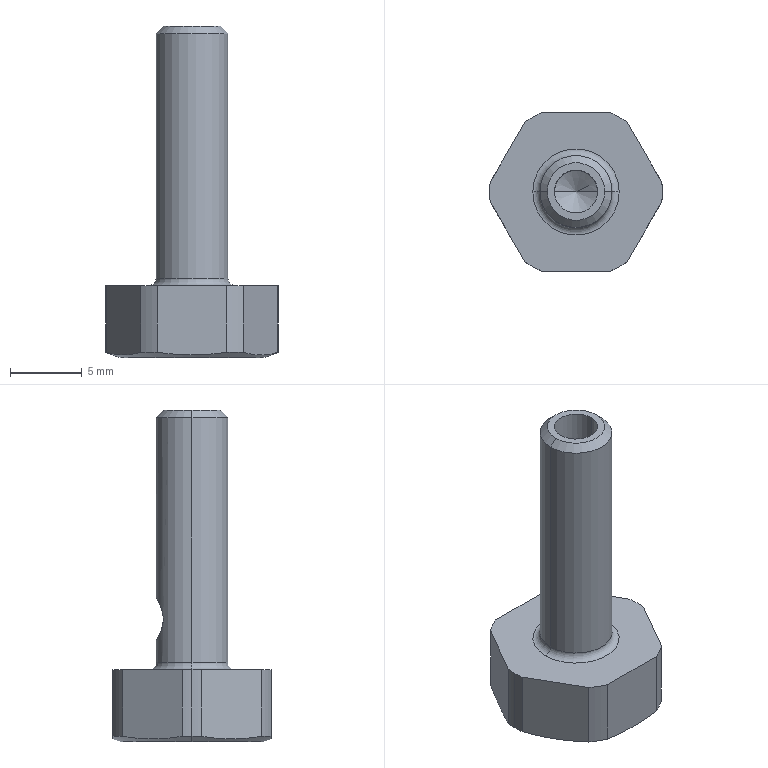Component | SolidWorks | 6.11-1937032107-0-2 | 1 solid | 32 faces | box 12 x 11 x 23 mm | volume 743 mm3 | cylinder 15 | plane 9 | cone 6 | torus 2 | commonest cylinder face diameters 12 x7 3 x6 5 x2 | material 40Cr
STEP:
#1=CARTESIAN_POINT('',(-0.09843,-1.772,-2.067));
#2=VERTEX_POINT('',#1);
#3=CARTESIAN_POINT('',(0.09843,-1.772,-2.067));
#4=VERTEX_POINT('',#3);
#5=CARTESIAN_POINT('',(0.,-1.772,-2.067));
#6=DIRECTION('',(0.,0.,1.));
#7=DIRECTION('',(1.,0.,0.));
#8=AXIS2_PLACEMENT_3D('',#5,#6,#7);
#9=CIRCLE('',#8,0.09843);
#10=EDGE_CURVE('',#2,#4,#9,.T.);
#11=ORIENTED_EDGE('',*,*,#10,.F.);
#12=CARTESIAN_POINT('',(-0.1181,-1.772,-2.087));
#13=VERTEX_POINT('',#12);
#14=CARTESIAN_POINT('',(-0.1181,-1.772,-2.067));
#15=DIRECTION('',(0.,1.,0.));
#16=DIRECTION('',(-1.,0.,0.));
#17=AXIS2_PLACEMENT_3D('',#14,#15,#16);
#18=CIRCLE('',#17,0.01969);
#19=EDGE_CURVE('',#2,#13,#18,.T.);
#20=ORIENTED_EDGE('',*,*,#19,.T.);
#21=CARTESIAN_POINT('',(0.1181,-1.772,-2.087));
#22=VERTEX_POINT('',#21);
#23=CARTESIAN_POINT('',(0.,-1.772,-2.087));
#24=DIRECTION('',(0.,0.,-1.));
#25=DIRECTION('',(1.,0.,0.));
#26=AXIS2_PLACEMENT_3D('',#23,#24,#25);
#27=CIRCLE('',#26,0.1181);
#28=EDGE_CURVE('',#22,#13,#27,.T.);
#29=ORIENTED_EDGE('',*,*,#28,.F.);
#30=CARTESIAN_POINT('',(0.1181,-1.772,-2.067));
#31=DIRECTION('',(0.,-1.,0.));
#32=DIRECTION('',(0.,0.,-1.));
#33=AXIS2_PLACEMENT_3D('',#30,#31,#32);
#34=CIRCLE('',#33,0.01969);
#35=EDGE_CURVE('',#4,#22,#34,.T.);
#36=ORIENTED_EDGE('',*,*,#35,.F.);
#37=EDGE_LOOP('',(#11,#20,#29,#36));
#38=FACE_OUTER_BOUND('',#37,.T.);
#39=CARTESIAN_POINT('',(0.,-1.772,-2.067));
#40=DIRECTION('',(0.,0.,1.));
#41=DIRECTION('',(1.,0.,0.));
#42=AXIS2_PLACEMENT_3D('',#39,#40,#41);
#43=TOROIDAL_SURFACE('',#42,0.1181,0.01969);
#44=ADVANCED_FACE('',(#38),#43,.F.);
#45=CARTESIAN_POINT('',(0.,-1.673,-1.89));
#46=VERTEX_POINT('',#45);
#47=CARTESIAN_POINT('',(0.,-1.673,-2.008));
#48=VERTEX_POINT('',#47);
#49=CARTESIAN_POINT('',(0.,-1.673,-1.89));
#50=CARTESIAN_POINT('',(-0.003988,-1.673,-1.89));
#51=CARTESIAN_POINT('',(-0.00791,-1.673,-1.89));
#52=CARTESIAN_POINT('',(-0.01563,-1.674,-1.892));
#53=CARTESIAN_POINT('',(-0.01942,-1.675,-1.893));
#54=CARTESIAN_POINT('',(-0.03011,-1.678,-1.897));
#55=CARTESIAN_POINT('',(-0.03651,-1.68,-1.902));
#56=CARTESIAN_POINT('',(-0.04449,-1.684,-1.91));
#57=CARTESIAN_POINT('',(-0.04691,-1.685,-1.913));
#58=CARTESIAN_POINT('',(-0.05111,-1.688,-1.919));
#59=CARTESIAN_POINT('',(-0.05291,-1.689,-1.922));
#60=CARTESIAN_POINT('',(-0.0559,-1.691,-1.929));
#61=CARTESIAN_POINT('',(-0.05707,-1.691,-1.933));
#62=CARTESIAN_POINT('',(-0.05864,-1.693,-1.941));
#63=CARTESIAN_POINT('',(-0.05905,-1.693,-1.945));
#64=CARTESIAN_POINT('',(-0.05906,-1.693,-1.957));
#65=CARTESIAN_POINT('',(-0.05742,-1.692,-1.965));
#66=CARTESIAN_POINT('',(-0.05294,-1.689,-1.975));
#67=CARTESIAN_POINT('',(-0.0511,-1.687,-1.979));
#68=CARTESIAN_POINT('',(-0.04688,-1.685,-1.985));
#69=CARTESIAN_POINT('',(-0.0445,-1.684,-1.988));
#70=CARTESIAN_POINT('',(-0.03645,-1.68,-1.996));
#71=CARTESIAN_POINT('',(-0.03014,-1.678,-2.));
#72=CARTESIAN_POINT('',(-0.0194,-1.675,-2.005));
#73=CARTESIAN_POINT('',(-0.01569,-1.674,-2.006));
#74=CARTESIAN_POINT('',(-0.00802,-1.673,-2.007));
#75=CARTESIAN_POINT('',(-0.004002,-1.673,-2.008));
#76=CARTESIAN_POINT('',(0.,-1.673,-2.008));
#77=B_SPLINE_CURVE_WITH_KNOTS('',3,(#49,#50,#51,#52,#53,#54,#55,#56,#57,#58,#59,#60,#61,#62,#63,#64,#65,#66,#67,#68,#69,#70,#71,#72,#73,#74,#75,#76),.UNSPECIFIED.,.F.,.F.,(4,2,2,2,2,2,2,2,2,2,2,2,2,4),(0.004812,0.005113,0.005413,0.006013,0.006313,0.006613,0.006914,0.007214,0.007814,0.008114,0.008415,0.009015,0.009315,0.009615),.UNSPECIFIED.);
#78=EDGE_CURVE('',#46,#48,#77,.T.);
#79=ORIENTED_EDGE('',*,*,#78,.F.);
#80=CARTESIAN_POINT('',(0.,-1.713,-1.89));
#81=VERTEX_POINT('',#80);
#82=CARTESIAN_POINT('',(0.,-1.772,-1.89));
#83=DIRECTION('',(0.,-1.,0.));
#84=VECTOR('',#83,39.37);
#85=LINE('',#82,#84);
#86=EDGE_CURVE('',#46,#81,#85,.T.);
#87=ORIENTED_EDGE('',*,*,#86,.T.);
#88=CARTESIAN_POINT('',(-0.05906,-1.772,-1.949));
#89=VERTEX_POINT('',#88);
#90=CARTESIAN_POINT('',(-0.05906,-1.772,-1.949));
#91=CARTESIAN_POINT('',(-0.05906,-1.737,-1.914));
#92=CARTESIAN_POINT('',(-0.03459,-1.713,-1.89));
#93=CARTESIAN_POINT('',(0.,-1.713,-1.89));
#94=(BOUNDED_CURVE()B_SPLINE_CURVE(3,(#90,#91,#92,#93),.UNSPECIFIED.,.F.,.F.)B_SPLINE_CURVE_WITH_KNOTS((4,4),(4.712,6.283),.UNSPECIFIED.)CURVE()GEOMETRIC_REPRESENTATION_ITEM()RATIONAL_B_SPLINE_CURVE((1.,0.8047,0.8047,1.))REPRESENTATION_ITEM(''));
#95=EDGE_CURVE('',#89,#81,#94,.T.);
#96=ORIENTED_EDGE('',*,*,#95,.F.);
#97=CARTESIAN_POINT('',(0.,-1.713,-2.008));
#98=VERTEX_POINT('',#97);
#99=CARTESIAN_POINT('',(0.,-1.713,-2.008));
#100=CARTESIAN_POINT('',(-0.03459,-1.713,-2.008));
#101=CARTESIAN_POINT('',(-0.05906,-1.737,-1.983));
#102=CARTESIAN_POINT('',(-0.05906,-1.772,-1.949));
#103=(BOUNDED_CURVE()B_SPLINE_CURVE(3,(#99,#100,#101,#102),.UNSPECIFIED.,.F.,.F.)B_SPLINE_CURVE_WITH_KNOTS((4,4),(3.142,4.712),.UNSPECIFIED.)CURVE()GEOMETRIC_REPRESENTATION_ITEM()RATIONAL_B_SPLINE_CURVE((1.,0.8047,0.8047,1.))REPRESENTATION_ITEM(''));
#104=EDGE_CURVE('',#98,#89,#103,.T.);
#105=ORIENTED_EDGE('',*,*,#104,.F.);
#106=CARTESIAN_POINT('',(0.,-1.772,-2.008));
#107=DIRECTION('',(0.,-1.,0.));
#108=VECTOR('',#107,39.37);
#109=LINE('',#106,#108);
#110=EDGE_CURVE('',#48,#98,#109,.T.);
#111=ORIENTED_EDGE('',*,*,#110,.F.);
#112=EDGE_LOOP('',(#79,#87,#96,#105,#111));
#113=FACE_OUTER_BOUND('',#112,.T.);
#114=CARTESIAN_POINT('',(0.,-1.772,-1.949));
#115=DIRECTION('',(0.,-1.,0.));
#116=DIRECTION('',(0.,0.,-1.));
#117=AXIS2_PLACEMENT_3D('',#114,#115,#116);
#118=CYLINDRICAL_SURFACE('',#117,0.05906);
#119=ADVANCED_FACE('',(#113),#118,.F.);
#120=CARTESIAN_POINT('',(-0.05906,-1.772,-2.008));
#121=VERTEX_POINT('',#120);
#122=CARTESIAN_POINT('',(0.05906,-1.772,-2.008));
#123=VERTEX_POINT('',#122);
#124=CARTESIAN_POINT('',(0.,-1.772,-2.008));
#125=DIRECTION('',(0.,0.,1.));
#126=DIRECTION('',(1.,0.,0.));
#127=AXIS2_PLACEMENT_3D('',#124,#125,#126);
#128=CIRCLE('',#127,0.05906);
#129=EDGE_CURVE('',#121,#123,#128,.T.);
#130=ORIENTED_EDGE('',*,*,#129,.F.);
#131=CARTESIAN_POINT('',(-0.05906,-1.772,-1.378));
#132=DIRECTION('',(0.,0.,1.));
#133=VECTOR('',#132,39.37);
#134=LINE('',#131,#133);
#135=EDGE_CURVE('',#121,#89,#134,.T.);
#136=ORIENTED_EDGE('',*,*,#135,.T.);
#137=CARTESIAN_POINT('',(-0.05906,-1.772,-1.378));
#138=VERTEX_POINT('',#137);
#139=CARTESIAN_POINT('',(-0.05906,-1.772,-1.378));
#140=DIRECTION('',(0.,0.,1.));
#141=VECTOR('',#140,39.37);
#142=LINE('',#139,#141);
#143=EDGE_CURVE('',#89,#138,#142,.T.);
#144=ORIENTED_EDGE('',*,*,#143,.T.);
#145=CARTESIAN_POINT('',(0.05906,-1.772,-1.378));
#146=VERTEX_POINT('',#145);
#147=CARTESIAN_POINT('',(0.,-1.772,-1.378));
#148=DIRECTION('',(0.,0.,1.));
#149=DIRECTION('',(1.,0.,0.));
#150=AXIS2_PLACEMENT_3D('',#147,#148,#149);
#151=CIRCLE('',#150,0.05906);
#152=EDGE_CURVE('',#138,#146,#151,.T.);
#153=ORIENTED_EDGE('',*,*,#152,.T.);
#154=CARTESIAN_POINT('',(0.05906,-1.772,-1.949));
#155=VERTEX_POINT('',#154);
#156=CARTESIAN_POINT('',(0.05906,-1.772,-1.378));
#157=DIRECTION('',(0.,0.,1.));
#158=VECTOR('',#157,39.37);
#159=LINE('',#156,#158);
#160=EDGE_CURVE('',#155,#146,#159,.T.);
#161=ORIENTED_EDGE('',*,*,#160,.F.);
#162=CARTESIAN_POINT('',(0.05906,-1.772,-1.378));
#163=DIRECTION('',(0.,0.,1.));
#164=VECTOR('',#163,39.37);
#165=LINE('',#162,#164);
#166=EDGE_CURVE('',#123,#155,#165,.T.);
#167=ORIENTED_EDGE('',*,*,#166,.F.);
#168=EDGE_LOOP('',(#130,#136,#144,#153,#161,#167));
#169=FACE_OUTER_BOUND('',#168,.T.);
#170=CARTESIAN_POINT('',(0.,-1.772,-1.378));
#171=DIRECTION('',(0.,0.,1.));
#172=DIRECTION('',(1.,0.,0.));
#173=AXIS2_PLACEMENT_3D('',#170,#171,#172);
#174=CYLINDRICAL_SURFACE('',#173,0.05906);
#175=ADVANCED_FACE('',(#169),#174,.F.);
#176=ORIENTED_EDGE('',*,*,#135,.F.);
#177=CARTESIAN_POINT('',(0.,-1.772,-2.008));
#178=DIRECTION('',(0.,0.,1.));
#179=DIRECTION('',(1.,0.,0.));
#180=AXIS2_PLACEMENT_3D('',#177,#178,#179);
#181=CIRCLE('',#180,0.05906);
#182=EDGE_CURVE('',#98,#121,#181,.T.);
#183=ORIENTED_EDGE('',*,*,#182,.F.);
#184=ORIENTED_EDGE('',*,*,#104,.T.);
#185=EDGE_LOOP('',(#176,#183,#184));
#186=FACE_OUTER_BOUND('',#185,.T.);
#187=CARTESIAN_POINT('',(0.,-1.772,-1.378));
#188=DIRECTION('',(0.,0.,1.));
#189=DIRECTION('',(1.,0.,0.));
#190=AXIS2_PLACEMENT_3D('',#187,#188,#189);
#191=CYLINDRICAL_SURFACE('',#190,0.05906);
#192=ADVANCED_FACE('',(#186),#191,.F.);
#193=CARTESIAN_POINT('',(0.,-1.772,-2.008));
#194=DIRECTION('',(0.,0.,1.));
#195=DIRECTION('',(1.,0.,0.));
#196=AXIS2_PLACEMENT_3D('',#193,#194,#195);
#197=CIRCLE('',#196,0.05906);
#198=EDGE_CURVE('',#123,#98,#197,.T.);
#199=ORIENTED_EDGE('',*,*,#198,.F.);
#200=ORIENTED_EDGE('',*,*,#166,.T.);
#201=CARTESIAN_POINT('',(0.05906,-1.772,-1.949));
#202=CARTESIAN_POINT('',(0.05906,-1.737,-1.983));
#203=CARTESIAN_POINT('',(0.03459,-1.713,-2.008));
#204=CARTESIAN_POINT('',(0.,-1.713,-2.008));
#205=(BOUNDED_CURVE()B_SPLINE_CURVE(3,(#201,#202,#203,#204),.UNSPECIFIED.,.F.,.F.)B_SPLINE_CURVE_WITH_KNOTS((4,4),(1.571,3.142),.UNSPECIFIED.)CURVE()GEOMETRIC_REPRESENTATION_ITEM()RATIONAL_B_SPLINE_CURVE((1.,0.8047,0.8047,1.))REPRESENTATION_ITEM(''));
#206=EDGE_CURVE('',#155,#98,#205,.T.);
#207=ORIENTED_EDGE('',*,*,#206,.T.);
#208=EDGE_LOOP('',(#199,#200,#207));
#209=FACE_OUTER_BOUND('',#208,.T.);
#210=CARTESIAN_POINT('',(0.,-1.772,-1.378));
#211=DIRECTION('',(0.,0.,1.));
#212=DIRECTION('',(1.,0.,0.));
#213=AXIS2_PLACEMENT_3D('',#210,#211,#212);
#214=CYLINDRICAL_SURFACE('',#213,0.05906);
#215=ADVANCED_FACE('',(#209),#214,.F.);
#216=CARTESIAN_POINT('',(-0.,-1.772,-2.043));
#217=VERTEX_POINT('',#216);
#218=CARTESIAN_POINT('',(0.05906,-1.772,-2.008));
#219=DIRECTION('',(0.8572,0.,0.515));
#220=VECTOR('',#219,39.37);
#221=LINE('',#218,#220);
#222=EDGE_CURVE('',#217,#123,#221,.T.);
#223=ORIENTED_EDGE('',*,*,#222,.F.);
#224=CARTESIAN_POINT('',(-0.05906,-1.772,-2.008));
#225=DIRECTION('',(-0.8572,0.,0.515));
#226=VECTOR('',#225,39.37);
#227=LINE('',#224,#226);
#228=EDGE_CURVE('',#217,#121,#227,.T.);
#229=ORIENTED_EDGE('',*,*,#228,.T.);
#230=ORIENTED_EDGE('',*,*,#129,.T.);
#231=EDGE_LOOP('',(#223,#229,#230));
#232=FACE_OUTER_BOUND('',#231,.T.);
#233=CARTESIAN_POINT('',(0.,-1.772,-2.008));
#234=DIRECTION('',(0.,0.,1.));
#235=DIRECTION('',(1.,0.,0.));
#236=AXIS2_PLACEMENT_3D('',#233,#234,#235);
#237=CONICAL_SURFACE('',#236,0.05906,1.03);
#238=ADVANCED_FACE('',(#232),#237,.F.);
#239=CARTESIAN_POINT('',(0.07874,-1.772,-1.378));
#240=VERTEX_POINT('',#239);
#241=CARTESIAN_POINT('',(-0.07874,-1.772,-1.378));
#242=VERTEX_POINT('',#241);
#243=CARTESIAN_POINT('',(0.,-1.772,-1.378));
#244=DIRECTION('',(0.,0.,1.));
#245=DIRECTION('',(1.,0.,0.));
#246=AXIS2_PLACEMENT_3D('',#243,#244,#245);
#247=CIRCLE('',#246,0.07874);
#248=EDGE_CURVE('',#240,#242,#247,.T.);
#249=ORIENTED_EDGE('',*,*,#248,.F.);
#250=CARTESIAN_POINT('',(0.09843,-1.772,-1.398));
#251=VERTEX_POINT('',#250);
#252=CARTESIAN_POINT('',(0.07874,-1.772,-1.378));
#253=DIRECTION('',(0.7071,0.,-0.7071));
#254=VECTOR('',#253,39.37);
#255=LINE('',#252,#254);
#256=EDGE_CURVE('',#240,#251,#255,.T.);
#257=ORIENTED_EDGE('',*,*,#256,.T.);
#258=CARTESIAN_POINT('',(-0.09843,-1.772,-1.398));
#259=VERTEX_POINT('',#258);
#260=CARTESIAN_POINT('',(0.,-1.772,-1.398));
#261=DIRECTION('',(0.,0.,-1.));
#262=DIRECTION('',(1.,0.,0.));
#263=AXIS2_PLACEMENT_3D('',#260,#261,#262);
#264=CIRCLE('',#263,0.09843);
#265=EDGE_CURVE('',#259,#251,#264,.T.);
#266=ORIENTED_EDGE('',*,*,#265,.F.);
#267=CARTESIAN_POINT('',(-0.07874,-1.772,-1.378));
#268=DIRECTION('',(-0.7071,0.,-0.7071));
#269=VECTOR('',#268,39.37);
#270=LINE('',#267,#269);
#271=EDGE_CURVE('',#242,#259,#270,.T.);
#272=ORIENTED_EDGE('',*,*,#271,.F.);
#273=EDGE_LOOP('',(#249,#257,#266,#272));
#274=FACE_OUTER_BOUND('',#273,.T.);
#275=CARTESIAN_POINT('',(0.,-1.772,-1.378));
#276=DIRECTION('',(0.,0.,-1.));
#277=DIRECTION('',(-1.,0.,0.));
#278=AXIS2_PLACEMENT_3D('',#275,#276,#277);
#279=CONICAL_SURFACE('',#278,0.07874,0.7854);
#280=ADVANCED_FACE('',(#274),#279,.T.);
#281=CARTESIAN_POINT('',(0.,-1.673,-2.008));
#282=CARTESIAN_POINT('',(0.00401,-1.673,-2.008));
#283=CARTESIAN_POINT('',(0.007935,-1.673,-2.007));
#284=CARTESIAN_POINT('',(0.01563,-1.674,-2.006));
#285=CARTESIAN_POINT('',(0.01943,-1.675,-2.005));
#286=CARTESIAN_POINT('',(0.03012,-1.678,-2.));
#287=CARTESIAN_POINT('',(0.03653,-1.68,-1.996));
#288=CARTESIAN_POINT('',(0.04714,-1.685,-1.985));
#289=CARTESIAN_POINT('',(0.05143,-1.688,-1.979));
#290=CARTESIAN_POINT('',(0.05738,-1.692,-1.965));
#291=CARTESIAN_POINT('',(0.05905,-1.693,-1.957));
#292=CARTESIAN_POINT('',(0.05906,-1.693,-1.945));
#293=CARTESIAN_POINT('',(0.05866,-1.693,-1.941));
#294=CARTESIAN_POINT('',(0.05709,-1.691,-1.933));
#295=CARTESIAN_POINT('',(0.05592,-1.691,-1.929));
#296=CARTESIAN_POINT('',(0.05144,-1.688,-1.919));
#297=CARTESIAN_POINT('',(0.04715,-1.685,-1.912));
#298=CARTESIAN_POINT('',(0.03648,-1.68,-1.902));
#299=CARTESIAN_POINT('',(0.03016,-1.678,-1.897));
#300=CARTESIAN_POINT('',(0.0158,-1.674,-1.891));
#301=CARTESIAN_POINT('',(0.007993,-1.673,-1.89));
#302=CARTESIAN_POINT('',(0.,-1.673,-1.89));
#303=B_SPLINE_CURVE_WITH_KNOTS('',3,(#281,#282,#283,#284,#285,#286,#287,#288,#289,#290,#291,#292,#293,#294,#295,#296,#297,#298,#299,#300,#301,#302),.UNSPECIFIED.,.F.,.F.,(4,2,2,2,2,2,2,2,2,2,4),(0.,0.0003008,0.0006015,0.001203,0.001805,0.002406,0.002707,0.003008,0.003609,0.004211,0.004812),.UNSPECIFIED.);
#304=EDGE_CURVE('',#48,#46,#303,.T.);
#305=ORIENTED_EDGE('',*,*,#304,.T.);
#306=ORIENTED_EDGE('',*,*,#78,.T.);
#307=EDGE_LOOP('',(#305,#306));
#308=FACE_BOUND('',#307,.T.);
#309=ORIENTED_EDGE('',*,*,#265,.T.);
#310=CARTESIAN_POINT('',(0.09843,-1.772,-1.378));
#311=DIRECTION('',(0.,0.,-1.));
#312=VECTOR('',#311,39.37);
#313=LINE('',#310,#312);
#314=EDGE_CURVE('',#251,#4,#313,.T.);
#315=ORIENTED_EDGE('',*,*,#314,.T.);
#316=CARTESIAN_POINT('',(0.,-1.772,-2.067));
#317=DIRECTION('',(0.,0.,1.));
#318=DIRECTION('',(1.,0.,0.));
#319=AXIS2_PLACEMENT_3D('',#316,#317,#318);
#320=CIRCLE('',#319,0.09843);
#321=EDGE_CURVE('',#4,#2,#320,.T.);
#322=ORIENTED_EDGE('',*,*,#321,.T.);
#323=CARTESIAN_POINT('',(-0.09843,-1.772,-1.378));
#324=DIRECTION('',(0.,0.,-1.));
#325=VECTOR('',#324,39.37);
#326=LINE('',#323,#325);
#327=EDGE_CURVE('',#259,#2,#326,.T.);
#328=ORIENTED_EDGE('',*,*,#327,.F.);
#329=EDGE_LOOP('',(#309,#315,#322,#328));
#330=FACE_OUTER_BOUND('',#329,.T.);
#331=CARTESIAN_POINT('',(0.,-1.772,-1.378));
#332=DIRECTION('',(0.,0.,-1.));
#333=DIRECTION('',(-1.,0.,0.));
#334=AXIS2_PLACEMENT_3D('',#331,#332,#333);
#335=CYLINDRICAL_SURFACE('',#334,0.09843);
#336=ADVANCED_FACE('',(#308,#330),#335,.T.);
#337=CARTESIAN_POINT('',(-0.1969,-1.772,-2.283));
#338=VERTEX_POINT('',#337);
#339=CARTESIAN_POINT('',(0.1969,-1.772,-2.283));
#340=VERTEX_POINT('',#339);
#341=CARTESIAN_POINT('',(0.,-1.772,-2.283));
#342=DIRECTION('',(0.,0.,-1.));
#343=DIRECTION('',(1.,0.,0.));
#344=AXIS2_PLACEMENT_3D('',#341,#342,#343);
#345=CIRCLE('',#344,0.1969);
#346=EDGE_CURVE('',#338,#340,#345,.T.);
#347=ORIENTED_EDGE('',*,*,#346,.F.);
#348=CARTESIAN_POINT('',(-0.2362,-1.772,-2.269));
#349=VERTEX_POINT('',#348);
#350=CARTESIAN_POINT('',(-0.2362,-1.772,-2.269));
#351=DIRECTION('',(-0.9397,0.,0.342));
#352=VECTOR('',#351,39.37);
#353=LINE('',#350,#352);
#354=EDGE_CURVE('',#338,#349,#353,.T.);
#355=ORIENTED_EDGE('',*,*,#354,.T.);
#356=CARTESIAN_POINT('',(-0.2347,-1.745,-2.269));
#357=VERTEX_POINT('',#356);
#358=CARTESIAN_POINT('',(0.,-1.772,-2.269));
#359=DIRECTION('',(0.,0.,1.));
#360=DIRECTION('',(1.,0.,0.));
#361=AXIS2_PLACEMENT_3D('',#358,#359,#360);
#362=CIRCLE('',#361,0.2362);
#363=EDGE_CURVE('',#357,#349,#362,.T.);
#364=ORIENTED_EDGE('',*,*,#363,.F.);
#365=CARTESIAN_POINT('',(-0.1403,-1.582,-2.269));
#366=VERTEX_POINT('',#365);
#367=CARTESIAN_POINT('',(-0.2347,-1.745,-2.269));
#368=CARTESIAN_POINT('',(-0.219,-1.718,-2.274));
#369=CARTESIAN_POINT('',(-0.1875,-1.663,-2.279));
#370=CARTESIAN_POINT('',(-0.1561,-1.609,-2.274));
#371=CARTESIAN_POINT('',(-0.1403,-1.582,-2.269));
#372=B_SPLINE_CURVE_WITH_KNOTS('',3,(#367,#368,#369,#370,#371),.UNSPECIFIED.,.F.,.F.,(4,1,4),(0.00000137,0.002399,0.004797),.UNSPECIFIED.);
#373=EDGE_CURVE('',#357,#366,#372,.T.);
#374=ORIENTED_EDGE('',*,*,#373,.T.);
#375=CARTESIAN_POINT('',(-0.09441,-1.555,-2.269));
#376=VERTEX_POINT('',#375);
#377=CARTESIAN_POINT('',(0.,-1.772,-2.269));
#378=DIRECTION('',(0.,0.,1.));
#379=DIRECTION('',(1.,0.,0.));
#380=AXIS2_PLACEMENT_3D('',#377,#378,#379);
#381=CIRCLE('',#380,0.2362);
#382=EDGE_CURVE('',#376,#366,#381,.T.);
#383=ORIENTED_EDGE('',*,*,#382,.F.);
#384=CARTESIAN_POINT('',(0.09441,-1.555,-2.269));
#385=VERTEX_POINT('',#384);
#386=CARTESIAN_POINT('',(-0.09441,-1.555,-2.269));
#387=CARTESIAN_POINT('',(-0.06285,-1.555,-2.274));
#388=CARTESIAN_POINT('',(-0.03131,-1.555,-2.276));
#389=CARTESIAN_POINT('',(0.03163,-1.555,-2.276));
#390=CARTESIAN_POINT('',(0.06304,-1.555,-2.274));
#391=CARTESIAN_POINT('',(0.09441,-1.555,-2.269));
#392=B_SPLINE_CURVE_WITH_KNOTS('',3,(#386,#387,#388,#389,#390,#391),.UNSPECIFIED.,.F.,.F.,(4,2,4),(0.006157,0.008575,0.01099),.UNSPECIFIED.);
#393=EDGE_CURVE('',#376,#385,#392,.T.);
#394=ORIENTED_EDGE('',*,*,#393,.T.);
#395=CARTESIAN_POINT('',(0.1403,-1.582,-2.269));
#396=VERTEX_POINT('',#395);
#397=CARTESIAN_POINT('',(0.,-1.772,-2.269));
#398=DIRECTION('',(0.,0.,1.));
#399=DIRECTION('',(1.,0.,0.));
#400=AXIS2_PLACEMENT_3D('',#397,#398,#399);
#401=CIRCLE('',#400,0.2362);
#402=EDGE_CURVE('',#396,#385,#401,.T.);
#403=ORIENTED_EDGE('',*,*,#402,.F.);
#404=CARTESIAN_POINT('',(0.2347,-1.745,-2.269));
#405=VERTEX_POINT('',#404);
#406=CARTESIAN_POINT('',(0.1403,-1.582,-2.269));
#407=CARTESIAN_POINT('',(0.1561,-1.609,-2.274));
#408=CARTESIAN_POINT('',(0.1875,-1.663,-2.279));
#409=CARTESIAN_POINT('',(0.219,-1.718,-2.274));
#410=CARTESIAN_POINT('',(0.2347,-1.745,-2.269));
#411=B_SPLINE_CURVE_WITH_KNOTS('',3,(#406,#407,#408,#409,#410),.UNSPECIFIED.,.F.,.F.,(4,1,4),(0.00000137,0.002399,0.004797),.UNSPECIFIED.);
#412=EDGE_CURVE('',#396,#405,#411,.T.);
#413=ORIENTED_EDGE('',*,*,#412,.T.);
#414=CARTESIAN_POINT('',(0.2362,-1.772,-2.269));
#415=VERTEX_POINT('',#414);
#416=CARTESIAN_POINT('',(0.,-1.772,-2.269));
#417=DIRECTION('',(0.,0.,1.));
#418=DIRECTION('',(1.,0.,0.));
#419=AXIS2_PLACEMENT_3D('',#416,#417,#418);
#420=CIRCLE('',#419,0.2362);
#421=EDGE_CURVE('',#415,#405,#420,.T.);
#422=ORIENTED_EDGE('',*,*,#421,.F.);
#423=CARTESIAN_POINT('',(0.2362,-1.772,-2.269));
#424=DIRECTION('',(0.9397,0.,0.342));
#425=VECTOR('',#424,39.37);
#426=LINE('',#423,#425);
#427=EDGE_CURVE('',#340,#415,#426,.T.);
#428=ORIENTED_EDGE('',*,*,#427,.F.);
#429=EDGE_LOOP('',(#347,#355,#364,#374,#383,#394,#403,#413,#422,#428));
#430=FACE_OUTER_BOUND('',#429,.T.);
#431=CARTESIAN_POINT('',(0.,-1.772,-2.269));
#432=DIRECTION('',(0.,0.,1.));
#433=DIRECTION('',(1.,0.,0.));
#434=AXIS2_PLACEMENT_3D('',#431,#432,#433);
#435=CONICAL_SURFACE('',#434,0.2362,1.222);
#436=ADVANCED_FACE('',(#430),#435,.T.);
#437=CARTESIAN_POINT('',(-0.2362,-1.772,-2.087));
#438=VERTEX_POINT('',#437);
#439=CARTESIAN_POINT('',(-0.2347,-1.798,-2.087));
#440=VERTEX_POINT('',#439);
#441=CARTESIAN_POINT('',(0.,-1.772,-2.087));
#442=DIRECTION('',(0.,0.,1.));
#443=DIRECTION('',(1.,0.,0.));
#444=AXIS2_PLACEMENT_3D('',#441,#442,#443);
#445=CIRCLE('',#444,0.2362);
#446=EDGE_CURVE('',#438,#440,#445,.T.);
#447=ORIENTED_EDGE('',*,*,#446,.F.);
#448=CARTESIAN_POINT('',(-0.2362,-1.772,-2.087));
#449=DIRECTION('',(0.,0.,-1.));
#450=VECTOR('',#449,39.37);
#451=LINE('',#448,#450);
#452=EDGE_CURVE('',#438,#349,#451,.T.);
#453=ORIENTED_EDGE('',*,*,#452,.T.);
#454=CARTESIAN_POINT('',(-0.2347,-1.798,-2.269));
#455=VERTEX_POINT('',#454);
#456=CARTESIAN_POINT('',(0.,-1.772,-2.269));
#457=DIRECTION('',(0.,0.,1.));
#458=DIRECTION('',(1.,0.,0.));
#459=AXIS2_PLACEMENT_3D('',#456,#457,#458);
#460=CIRCLE('',#459,0.2362);
#461=EDGE_CURVE('',#349,#455,#460,.T.);
#462=ORIENTED_EDGE('',*,*,#461,.T.);
#463=CARTESIAN_POINT('',(-0.2347,-1.798,-2.087));
#464=DIRECTION('',(0.,0.,-1.));
#465=VECTOR('',#464,39.37);
#466=LINE('',#463,#465);
#467=EDGE_CURVE('',#440,#455,#466,.T.);
#468=ORIENTED_EDGE('',*,*,#467,.F.);
#469=EDGE_LOOP('',(#447,#453,#462,#468));
#470=FACE_OUTER_BOUND('',#469,.T.);
#471=CARTESIAN_POINT('',(0.,-1.772,-2.087));
#472=DIRECTION('',(0.,0.,-1.));
#473=DIRECTION('',(-1.,0.,0.));
#474=AXIS2_PLACEMENT_3D('',#471,#472,#473);
#475=CYLINDRICAL_SURFACE('',#474,0.2362);
#476=ADVANCED_FACE('',(#470),#475,.T.);
#477=ORIENTED_EDGE('',*,*,#28,.T.);
#478=CARTESIAN_POINT('',(0.,-1.772,-2.087));
#479=DIRECTION('',(0.,0.,-1.));
#480=DIRECTION('',(1.,0.,0.));
#481=AXIS2_PLACEMENT_3D('',#478,#479,#480);
#482=CIRCLE('',#481,0.1181);
#483=EDGE_CURVE('',#13,#22,#482,.T.);
#484=ORIENTED_EDGE('',*,*,#483,.T.);
#485=EDGE_LOOP('',(#477,#484));
#486=FACE_BOUND('',#485,.T.);
#487=CARTESIAN_POINT('',(-0.2347,-1.745,-2.087));
#488=VERTEX_POINT('',#487);
#489=CARTESIAN_POINT('',(0.,-1.772,-2.087));
#490=DIRECTION('',(0.,0.,1.));
#491=DIRECTION('',(1.,0.,0.));
#492=AXIS2_PLACEMENT_3D('',#489,#490,#491);
#493=CIRCLE('',#492,0.2362);
#494=EDGE_CURVE('',#488,#438,#493,.T.);
#495=ORIENTED_EDGE('',*,*,#494,.T.);
#496=ORIENTED_EDGE('',*,*,#446,.T.);
#497=CARTESIAN_POINT('',(-0.1403,-1.962,-2.087));
#498=VERTEX_POINT('',#497);
#499=CARTESIAN_POINT('',(-0.1875,-1.88,-2.087));
#500=DIRECTION('',(0.5,-0.866,0.));
#501=VECTOR('',#500,39.37);
#502=LINE('',#499,#501);
#503=EDGE_CURVE('',#440,#498,#502,.T.);
#504=ORIENTED_EDGE('',*,*,#503,.T.);
#505=CARTESIAN_POINT('',(-0.09441,-1.988,-2.087));
#506=VERTEX_POINT('',#505);
#507=CARTESIAN_POINT('',(0.,-1.772,-2.087));
#508=DIRECTION('',(0.,0.,1.));
#509=DIRECTION('',(1.,0.,0.));
#510=AXIS2_PLACEMENT_3D('',#507,#508,#509);
#511=CIRCLE('',#510,0.2362);
#512=EDGE_CURVE('',#498,#506,#511,.T.);
#513=ORIENTED_EDGE('',*,*,#512,.T.);
#514=CARTESIAN_POINT('',(0.09441,-1.988,-2.087));
#515=VERTEX_POINT('',#514);
#516=CARTESIAN_POINT('',(0.,-1.988,-2.087));
#517=DIRECTION('',(1.,0.,0.));
#518=VECTOR('',#517,39.37);
#519=LINE('',#516,#518);
#520=EDGE_CURVE('',#506,#515,#519,.T.);
#521=ORIENTED_EDGE('',*,*,#520,.T.);
#522=CARTESIAN_POINT('',(0.1403,-1.962,-2.087));
#523=VERTEX_POINT('',#522);
#524=CARTESIAN_POINT('',(0.,-1.772,-2.087));
#525=DIRECTION('',(0.,0.,1.));
#526=DIRECTION('',(1.,0.,0.));
#527=AXIS2_PLACEMENT_3D('',#524,#525,#526);
#528=CIRCLE('',#527,0.2362);
#529=EDGE_CURVE('',#515,#523,#528,.T.);
#530=ORIENTED_EDGE('',*,*,#529,.T.);
#531=CARTESIAN_POINT('',(0.2347,-1.798,-2.087));
#532=VERTEX_POINT('',#531);
#533=CARTESIAN_POINT('',(0.1875,-1.88,-2.087));
#534=DIRECTION('',(0.5,0.866,0.));
#535=VECTOR('',#534,39.37);
#536=LINE('',#533,#535);
#537=EDGE_CURVE('',#523,#532,#536,.T.);
#538=ORIENTED_EDGE('',*,*,#537,.T.);
#539=CARTESIAN_POINT('',(0.2347,-1.745,-2.087));
#540=VERTEX_POINT('',#539);
#541=CARTESIAN_POINT('',(0.,-1.772,-2.087));
#542=DIRECTION('',(0.,0.,1.));
#543=DIRECTION('',(1.,0.,0.));
#544=AXIS2_PLACEMENT_3D('',#541,#542,#543);
#545=CIRCLE('',#544,0.2362);
#546=EDGE_CURVE('',#532,#540,#545,.T.);
#547=ORIENTED_EDGE('',*,*,#546,.T.);
#548=CARTESIAN_POINT('',(0.1403,-1.582,-2.087));
#549=VERTEX_POINT('',#548);
#550=CARTESIAN_POINT('',(0.1875,-1.663,-2.087));
#551=DIRECTION('',(-0.5,0.866,0.));
#552=VECTOR('',#551,39.37);
#553=LINE('',#550,#552);
#554=EDGE_CURVE('',#540,#549,#553,.T.);
#555=ORIENTED_EDGE('',*,*,#554,.T.);
#556=CARTESIAN_POINT('',(0.09441,-1.555,-2.087));
#557=VERTEX_POINT('',#556);
#558=CARTESIAN_POINT('',(0.,-1.772,-2.087));
#559=DIRECTION('',(0.,0.,1.));
#560=DIRECTION('',(1.,0.,0.));
#561=AXIS2_PLACEMENT_3D('',#558,#559,#560);
#562=CIRCLE('',#561,0.2362);
#563=EDGE_CURVE('',#549,#557,#562,.T.);
#564=ORIENTED_EDGE('',*,*,#563,.T.);
#565=CARTESIAN_POINT('',(-0.09441,-1.555,-2.087));
#566=VERTEX_POINT('',#565);
#567=CARTESIAN_POINT('',(0.,-1.555,-2.087));
#568=DIRECTION('',(-1.,0.,0.));
#569=VECTOR('',#568,39.37);
#570=LINE('',#567,#569);
#571=EDGE_CURVE('',#557,#566,#570,.T.);
#572=ORIENTED_EDGE('',*,*,#571,.T.);
#573=CARTESIAN_POINT('',(-0.1403,-1.582,-2.087));
#574=VERTEX_POINT('',#573);
#575=CARTESIAN_POINT('',(0.,-1.772,-2.087));
#576=DIRECTION('',(0.,0.,1.));
#577=DIRECTION('',(1.,0.,0.));
#578=AXIS2_PLACEMENT_3D('',#575,#576,#577);
#579=CIRCLE('',#578,0.2362);
#580=EDGE_CURVE('',#566,#574,#579,.T.);
#581=ORIENTED_EDGE('',*,*,#580,.T.);
#582=CARTESIAN_POINT('',(-0.1875,-1.663,-2.087));
#583=DIRECTION('',(-0.5,-0.866,0.));
#584=VECTOR('',#583,39.37);
#585=LINE('',#582,#584);
#586=EDGE_CURVE('',#574,#488,#585,.T.);
#587=ORIENTED_EDGE('',*,*,#586,.T.);
#588=EDGE_LOOP('',(#495,#496,#504,#513,#521,#530,#538,#547,#555,#564,#572,#581,#587));
#589=FACE_OUTER_BOUND('',#588,.T.);
#590=CARTESIAN_POINT('',(0.,-1.772,-2.087));
#591=DIRECTION('',(0.,0.,1.));
#592=DIRECTION('',(1.,0.,0.));
#593=AXIS2_PLACEMENT_3D('',#590,#591,#592);
#594=PLANE('',#593);
#595=ADVANCED_FACE('',(#486,#589),#594,.T.);
#596=ORIENTED_EDGE('',*,*,#452,.F.);
#597=ORIENTED_EDGE('',*,*,#494,.F.);
#598=CARTESIAN_POINT('',(-0.2347,-1.745,-2.087));
#599=DIRECTION('',(0.,0.,1.));
#600=VECTOR('',#599,39.37);
#601=LINE('',#598,#600);
#602=EDGE_CURVE('',#357,#488,#601,.T.);
#603=ORIENTED_EDGE('',*,*,#602,.F.);
#604=ORIENTED_EDGE('',*,*,#363,.T.);
#605=EDGE_LOOP('',(#596,#597,#603,#604));
#606=FACE_OUTER_BOUND('',#605,.T.);
#607=CARTESIAN_POINT('',(0.,-1.772,-2.087));
#608=DIRECTION('',(0.,0.,-1.));
#609=DIRECTION('',(-1.,0.,0.));
#610=AXIS2_PLACEMENT_3D('',#607,#608,#609);
#611=CYLINDRICAL_SURFACE('',#610,0.2362);
#612=ADVANCED_FACE('',(#606),#611,.T.);
#613=CARTESIAN_POINT('',(-0.1403,-1.962,-2.269));
#614=VERTEX_POINT('',#613);
#615=CARTESIAN_POINT('',(-0.1403,-1.962,-2.087));
#616=DIRECTION('',(0.,0.,1.));
#617=VECTOR('',#616,39.37);
#618=LINE('',#615,#617);
#619=EDGE_CURVE('',#614,#498,#618,.T.);
#620=ORIENTED_EDGE('',*,*,#619,.F.);
#621=CARTESIAN_POINT('',(-0.09441,-1.988,-2.269));
#622=VERTEX_POINT('',#621);
#623=CARTESIAN_POINT('',(0.,-1.772,-2.269));
#624=DIRECTION('',(0.,0.,1.));
#625=DIRECTION('',(1.,0.,0.));
#626=AXIS2_PLACEMENT_3D('',#623,#624,#625);
#627=CIRCLE('',#626,0.2362);
#628=EDGE_CURVE('',#614,#622,#627,.T.);
#629=ORIENTED_EDGE('',*,*,#628,.T.);
#630=CARTESIAN_POINT('',(-0.09441,-1.988,-2.087));
#631=DIRECTION('',(0.,0.,-1.));
#632=VECTOR('',#631,39.37);
#633=LINE('',#630,#632);
#634=EDGE_CURVE('',#506,#622,#633,.T.);
#635=ORIENTED_EDGE('',*,*,#634,.F.);
#636=ORIENTED_EDGE('',*,*,#512,.F.);
#637=EDGE_LOOP('',(#620,#629,#635,#636));
#638=FACE_OUTER_BOUND('',#637,.T.);
#639=CARTESIAN_POINT('',(0.,-1.772,-2.087));
#640=DIRECTION('',(0.,0.,-1.));
#641=DIRECTION('',(-1.,0.,0.));
#642=AXIS2_PLACEMENT_3D('',#639,#640,#641);
#643=CYLINDRICAL_SURFACE('',#642,0.2362);
#644=ADVANCED_FACE('',(#638),#643,.T.);
#645=CARTESIAN_POINT('',(0.09441,-1.988,-2.269));
#646=VERTEX_POINT('',#645);
#647=CARTESIAN_POINT('',(0.09441,-1.988,-2.087));
#648=DIRECTION('',(0.,0.,1.));
#649=VECTOR('',#648,39.37);
#650=LINE('',#647,#649);
#651=EDGE_CURVE('',#646,#515,#650,.T.);
#652=ORIENTED_EDGE('',*,*,#651,.F.);
#653=CARTESIAN_POINT('',(0.1403,-1.962,-2.269));
#654=VERTEX_POINT('',#653);
#655=CARTESIAN_POINT('',(0.,-1.772,-2.269));
#656=DIRECTION('',(0.,0.,1.));
#657=DIRECTION('',(1.,0.,0.));
#658=AXIS2_PLACEMENT_3D('',#655,#656,#657);
#659=CIRCLE('',#658,0.2362);
#660=EDGE_CURVE('',#646,#654,#659,.T.);
#661=ORIENTED_EDGE('',*,*,#660,.T.);
#662=CARTESIAN_POINT('',(0.1403,-1.962,-2.087));
#663=DIRECTION('',(0.,0.,-1.));
#664=VECTOR('',#663,39.37);
#665=LINE('',#662,#664);
#666=EDGE_CURVE('',#523,#654,#665,.T.);
#667=ORIENTED_EDGE('',*,*,#666,.F.);
#668=ORIENTED_EDGE('',*,*,#529,.F.);
#669=EDGE_LOOP('',(#652,#661,#667,#668));
#670=FACE_OUTER_BOUND('',#669,.T.);
#671=CARTESIAN_POINT('',(0.,-1.772,-2.087));
#672=DIRECTION('',(0.,0.,-1.));
#673=DIRECTION('',(-1.,0.,0.));
#674=AXIS2_PLACEMENT_3D('',#671,#672,#673);
#675=CYLINDRICAL_SURFACE('',#674,0.2362);
#676=ADVANCED_FACE('',(#670),#675,.T.);
#677=CARTESIAN_POINT('',(0.2347,-1.798,-2.269));
#678=VERTEX_POINT('',#677);
#679=CARTESIAN_POINT('',(0.2347,-1.798,-2.087));
#680=DIRECTION('',(0.,0.,1.));
#681=VECTOR('',#680,39.37);
#682=LINE('',#679,#681);
#683=EDGE_CURVE('',#678,#532,#682,.T.);
#684=ORIENTED_EDGE('',*,*,#683,.F.);
#685=CARTESIAN_POINT('',(0.,-1.772,-2.269));
#686=DIRECTION('',(0.,0.,1.));
#687=DIRECTION('',(1.,0.,0.));
#688=AXIS2_PLACEMENT_3D('',#685,#686,#687);
#689=CIRCLE('',#688,0.2362);
#690=EDGE_CURVE('',#678,#415,#689,.T.);
#691=ORIENTED_EDGE('',*,*,#690,.T.);
#692=ORIENTED_EDGE('',*,*,#421,.T.);
#693=CARTESIAN_POINT('',(0.2347,-1.745,-2.087));
#694=DIRECTION('',(0.,0.,-1.));
#695=VECTOR('',#694,39.37);
#696=LINE('',#693,#695);
#697=EDGE_CURVE('',#540,#405,#696,.T.);
#698=ORIENTED_EDGE('',*,*,#697,.F.);
#699=ORIENTED_EDGE('',*,*,#546,.F.);
#700=EDGE_LOOP('',(#684,#691,#692,#698,#699));
#701=FACE_OUTER_BOUND('',#700,.T.);
#702=CARTESIAN_POINT('',(0.,-1.772,-2.087));
#703=DIRECTION('',(0.,0.,-1.));
#704=DIRECTION('',(-1.,0.,0.));
#705=AXIS2_PLACEMENT_3D('',#702,#703,#704);
#706=CYLINDRICAL_SURFACE('',#705,0.2362);
#707=ADVANCED_FACE('',(#701),#706,.T.);
#708=CARTESIAN_POINT('',(0.1403,-1.582,-2.087));
#709=DIRECTION('',(0.,0.,1.));
#710=VECTOR('',#709,39.37);
#711=LINE('',#708,#710);
#712=EDGE_CURVE('',#396,#549,#711,.T.);
#713=ORIENTED_EDGE('',*,*,#712,.F.);
#714=ORIENTED_EDGE('',*,*,#402,.T.);
#715=CARTESIAN_POINT('',(0.09441,-1.555,-2.087));
#716=DIRECTION('',(0.,0.,-1.));
#717=VECTOR('',#716,39.37);
#718=LINE('',#715,#717);
#719=EDGE_CURVE('',#557,#385,#718,.T.);
#720=ORIENTED_EDGE('',*,*,#719,.F.);
#721=ORIENTED_EDGE('',*,*,#563,.F.);
#722=EDGE_LOOP('',(#713,#714,#720,#721));
#723=FACE_OUTER_BOUND('',#722,.T.);
#724=CARTESIAN_POINT('',(0.,-1.772,-2.087));
#725=DIRECTION('',(0.,0.,-1.));
#726=DIRECTION('',(-1.,0.,0.));
#727=AXIS2_PLACEMENT_3D('',#724,#725,#726);
#728=CYLINDRICAL_SURFACE('',#727,0.2362);
#729=ADVANCED_FACE('',(#723),#728,.T.);
#730=CARTESIAN_POINT('',(-0.09441,-1.555,-2.087));
#731=DIRECTION('',(0.,0.,1.));
#732=VECTOR('',#731,39.37);
#733=LINE('',#730,#732);
#734=EDGE_CURVE('',#376,#566,#733,.T.);
#735=ORIENTED_EDGE('',*,*,#734,.F.);
#736=ORIENTED_EDGE('',*,*,#382,.T.);
#737=CARTESIAN_POINT('',(-0.1403,-1.582,-2.087));
#738=DIRECTION('',(0.,0.,-1.));
#739=VECTOR('',#738,39.37);
#740=LINE('',#737,#739);
#741=EDGE_CURVE('',#574,#366,#740,.T.);
#742=ORIENTED_EDGE('',*,*,#741,.F.);
#743=ORIENTED_EDGE('',*,*,#580,.F.);
#744=EDGE_LOOP('',(#735,#736,#742,#743));
#745=FACE_OUTER_BOUND('',#744,.T.);
#746=CARTESIAN_POINT('',(0.,-1.772,-2.087));
#747=DIRECTION('',(0.,0.,-1.));
#748=DIRECTION('',(-1.,0.,0.));
#749=AXIS2_PLACEMENT_3D('',#746,#747,#748);
#750=CYLINDRICAL_SURFACE('',#749,0.2362);
#751=ADVANCED_FACE('',(#745),#750,.T.);
#752=ORIENTED_EDGE('',*,*,#354,.F.);
#753=CARTESIAN_POINT('',(0.,-1.772,-2.283));
#754=DIRECTION('',(0.,0.,-1.));
#755=DIRECTION('',(1.,0.,0.));
#756=AXIS2_PLACEMENT_3D('',#753,#754,#755);
#757=CIRCLE('',#756,0.1969);
#758=EDGE_CURVE('',#340,#338,#757,.T.);
#759=ORIENTED_EDGE('',*,*,#758,.F.);
#760=ORIENTED_EDGE('',*,*,#427,.T.);
#761=ORIENTED_EDGE('',*,*,#690,.F.);
#762=CARTESIAN_POINT('',(0.2347,-1.798,-2.269));
#763=CARTESIAN_POINT('',(0.219,-1.825,-2.274));
#764=CARTESIAN_POINT('',(0.1875,-1.88,-2.279));
#765=CARTESIAN_POINT('',(0.1561,-1.934,-2.274));
#766=CARTESIAN_POINT('',(0.1403,-1.962,-2.269));
#767=B_SPLINE_CURVE_WITH_KNOTS('',3,(#762,#763,#764,#765,#766),.UNSPECIFIED.,.F.,.F.,(4,1,4),(0.00000137,0.002399,0.004797),.UNSPECIFIED.);
#768=EDGE_CURVE('',#678,#654,#767,.T.);
#769=ORIENTED_EDGE('',*,*,#768,.T.);
#770=ORIENTED_EDGE('',*,*,#660,.F.);
#771=CARTESIAN_POINT('',(0.09441,-1.988,-2.269));
#772=CARTESIAN_POINT('',(0.06304,-1.988,-2.274));
#773=CARTESIAN_POINT('',(0.03163,-1.988,-2.276));
#774=CARTESIAN_POINT('',(-0.03131,-1.988,-2.276));
#775=CARTESIAN_POINT('',(-0.06285,-1.988,-2.274));
#776=CARTESIAN_POINT('',(-0.09441,-1.988,-2.269));
#777=B_SPLINE_CURVE_WITH_KNOTS('',3,(#771,#772,#773,#774,#775,#776),.UNSPECIFIED.,.F.,.F.,(4,2,4),(0.01226,0.01467,0.01709),.UNSPECIFIED.);
#778=EDGE_CURVE('',#646,#622,#777,.T.);
#779=ORIENTED_EDGE('',*,*,#778,.T.);
#780=ORIENTED_EDGE('',*,*,#628,.F.);
#781=CARTESIAN_POINT('',(-0.1403,-1.962,-2.269));
#782=CARTESIAN_POINT('',(-0.1561,-1.934,-2.274));
#783=CARTESIAN_POINT('',(-0.1875,-1.88,-2.279));
#784=CARTESIAN_POINT('',(-0.219,-1.825,-2.274));
#785=CARTESIAN_POINT('',(-0.2347,-1.798,-2.269));
#786=B_SPLINE_CURVE_WITH_KNOTS('',3,(#781,#782,#783,#784,#785),.UNSPECIFIED.,.F.,.F.,(4,1,4),(0.00000137,0.002399,0.004797),.UNSPECIFIED.);
#787=EDGE_CURVE('',#614,#455,#786,.T.);
#788=ORIENTED_EDGE('',*,*,#787,.T.);
#789=ORIENTED_EDGE('',*,*,#461,.F.);
#790=EDGE_LOOP('',(#752,#759,#760,#761,#769,#770,#779,#780,#788,#789));
#791=FACE_OUTER_BOUND('',#790,.T.);
#792=CARTESIAN_POINT('',(0.,-1.772,-2.269));
#793=DIRECTION('',(0.,0.,1.));
#794=DIRECTION('',(1.,0.,0.));
#795=AXIS2_PLACEMENT_3D('',#792,#793,#794);
#796=CONICAL_SURFACE('',#795,0.2362,1.222);
#797=ADVANCED_FACE('',(#791),#796,.T.);
#798=ORIENTED_EDGE('',*,*,#758,.T.);
#799=ORIENTED_EDGE('',*,*,#346,.T.);
#800=EDGE_LOOP('',(#798,#799));
#801=FACE_OUTER_BOUND('',#800,.T.);
#802=CARTESIAN_POINT('',(0.,-1.772,-2.283));
#803=DIRECTION('',(0.,0.,1.));
#804=DIRECTION('',(1.,0.,0.));
#805=AXIS2_PLACEMENT_3D('',#802,#803,#804);
#806=PLANE('',#805);
#807=ADVANCED_FACE('',(#801),#806,.F.);
#808=ORIENTED_EDGE('',*,*,#314,.F.);
#809=CARTESIAN_POINT('',(0.,-1.772,-1.398));
#810=DIRECTION('',(0.,0.,-1.));
#811=DIRECTION('',(1.,0.,0.));
#812=AXIS2_PLACEMENT_3D('',#809,#810,#811);
#813=CIRCLE('',#812,0.09843);
#814=EDGE_CURVE('',#251,#259,#813,.T.);
#815=ORIENTED_EDGE('',*,*,#814,.T.);
#816=ORIENTED_EDGE('',*,*,#327,.T.);
#817=ORIENTED_EDGE('',*,*,#10,.T.);
#818=EDGE_LOOP('',(#808,#815,#816,#817));
#819=FACE_OUTER_BOUND('',#818,.T.);
#820=CARTESIAN_POINT('',(0.,-1.772,-1.378));
#821=DIRECTION('',(0.,0.,-1.));
#822=DIRECTION('',(-1.,0.,0.));
#823=AXIS2_PLACEMENT_3D('',#820,#821,#822);
#824=CYLINDRICAL_SURFACE('',#823,0.09843);
#825=ADVANCED_FACE('',(#819),#824,.T.);
#826=CARTESIAN_POINT('',(0.,-1.772,-1.378));
#827=DIRECTION('',(0.,0.,1.));
#828=DIRECTION('',(1.,0.,0.));
#829=AXIS2_PLACEMENT_3D('',#826,#827,#828);
#830=CIRCLE('',#829,0.05906);
#831=EDGE_CURVE('',#146,#138,#830,.T.);
#832=ORIENTED_EDGE('',*,*,#831,.F.);
#833=ORIENTED_EDGE('',*,*,#152,.F.);
#834=EDGE_LOOP('',(#832,#833));
#835=FACE_BOUND('',#834,.T.);
#836=CARTESIAN_POINT('',(0.,-1.772,-1.378));
#837=DIRECTION('',(0.,0.,1.));
#838=DIRECTION('',(1.,0.,0.));
#839=AXIS2_PLACEMENT_3D('',#836,#837,#838);
#840=CIRCLE('',#839,0.07874);
#841=EDGE_CURVE('',#242,#240,#840,.T.);
#842=ORIENTED_EDGE('',*,*,#841,.T.);
#843=ORIENTED_EDGE('',*,*,#248,.T.);
#844=EDGE_LOOP('',(#842,#843));
#845=FACE_OUTER_BOUND('',#844,.T.);
#846=CARTESIAN_POINT('',(0.,-1.772,-1.378));
#847=DIRECTION('',(0.,0.,1.));
#848=DIRECTION('',(1.,0.,0.));
#849=AXIS2_PLACEMENT_3D('',#846,#847,#848);
#850=PLANE('',#849);
#851=ADVANCED_FACE('',(#835,#845),#850,.T.);
#852=ORIENTED_EDGE('',*,*,#741,.T.);
#853=ORIENTED_EDGE('',*,*,#373,.F.);
#854=ORIENTED_EDGE('',*,*,#602,.T.);
#855=ORIENTED_EDGE('',*,*,#586,.F.);
#856=EDGE_LOOP('',(#852,#853,#854,#855));
#857=FACE_OUTER_BOUND('',#856,.T.);
#858=CARTESIAN_POINT('',(-0.25,-1.772,-1.693));
#859=DIRECTION('',(-0.866,0.5,0.));
#860=DIRECTION('',(-0.5,-0.866,0.));
#861=AXIS2_PLACEMENT_3D('',#858,#859,#860);
#862=PLANE('',#861);
#863=ADVANCED_FACE('',(#857),#862,.T.);
#864=ORIENTED_EDGE('',*,*,#719,.T.);
#865=ORIENTED_EDGE('',*,*,#393,.F.);
#866=ORIENTED_EDGE('',*,*,#734,.T.);
#867=ORIENTED_EDGE('',*,*,#571,.F.);
#868=EDGE_LOOP('',(#864,#865,#866,#867));
#869=FACE_OUTER_BOUND('',#868,.T.);
#870=CARTESIAN_POINT('',(-0.125,-1.555,-1.693));
#871=DIRECTION('',(0.,1.,0.));
#872=DIRECTION('',(0.,0.,1.));
#873=AXIS2_PLACEMENT_3D('',#870,#871,#872);
#874=PLANE('',#873);
#875=ADVANCED_FACE('',(#869),#874,.T.);
#876=ORIENTED_EDGE('',*,*,#697,.T.);
#877=ORIENTED_EDGE('',*,*,#412,.F.);
#878=ORIENTED_EDGE('',*,*,#712,.T.);
#879=ORIENTED_EDGE('',*,*,#554,.F.);
#880=EDGE_LOOP('',(#876,#877,#878,#879));
#881=FACE_OUTER_BOUND('',#880,.T.);
#882=CARTESIAN_POINT('',(0.125,-1.555,-1.693));
#883=DIRECTION('',(0.866,0.5,0.));
#884=DIRECTION('',(-0.5,0.866,0.));
#885=AXIS2_PLACEMENT_3D('',#882,#883,#884);
#886=PLANE('',#885);
#887=ADVANCED_FACE('',(#881),#886,.T.);
#888=ORIENTED_EDGE('',*,*,#666,.T.);
#889=ORIENTED_EDGE('',*,*,#768,.F.);
#890=ORIENTED_EDGE('',*,*,#683,.T.);
#891=ORIENTED_EDGE('',*,*,#537,.F.);
#892=EDGE_LOOP('',(#888,#889,#890,#891));
#893=FACE_OUTER_BOUND('',#892,.T.);
#894=CARTESIAN_POINT('',(0.25,-1.772,-1.693));
#895=DIRECTION('',(0.866,-0.5,0.));
#896=DIRECTION('',(0.5,0.866,0.));
#897=AXIS2_PLACEMENT_3D('',#894,#895,#896);
#898=PLANE('',#897);
#899=ADVANCED_FACE('',(#893),#898,.T.);
#900=ORIENTED_EDGE('',*,*,#634,.T.);
#901=ORIENTED_EDGE('',*,*,#778,.F.);
#902=ORIENTED_EDGE('',*,*,#651,.T.);
#903=ORIENTED_EDGE('',*,*,#520,.F.);
#904=EDGE_LOOP('',(#900,#901,#902,#903));
#905=FACE_OUTER_BOUND('',#904,.T.);
#906=CARTESIAN_POINT('',(0.125,-1.988,-1.693));
#907=DIRECTION('',(0.,-1.,0.));
#908=DIRECTION('',(1.,0.,0.));
#909=AXIS2_PLACEMENT_3D('',#906,#907,#908);
#910=PLANE('',#909);
#911=ADVANCED_FACE('',(#905),#910,.T.);
#912=ORIENTED_EDGE('',*,*,#467,.T.);
#913=ORIENTED_EDGE('',*,*,#787,.F.);
#914=ORIENTED_EDGE('',*,*,#619,.T.);
#915=ORIENTED_EDGE('',*,*,#503,.F.);
#916=EDGE_LOOP('',(#912,#913,#914,#915));
#917=FACE_OUTER_BOUND('',#916,.T.);
#918=CARTESIAN_POINT('',(-0.125,-1.988,-1.693));
#919=DIRECTION('',(-0.866,-0.5,0.));
#920=DIRECTION('',(0.5,-0.866,0.));
#921=AXIS2_PLACEMENT_3D('',#918,#919,#920);
#922=PLANE('',#921);
#923=ADVANCED_FACE('',(#917),#922,.T.);
#924=ORIENTED_EDGE('',*,*,#256,.F.);
#925=ORIENTED_EDGE('',*,*,#841,.F.);
#926=ORIENTED_EDGE('',*,*,#271,.T.);
#927=ORIENTED_EDGE('',*,*,#814,.F.);
#928=EDGE_LOOP('',(#924,#925,#926,#927));
#929=FACE_OUTER_BOUND('',#928,.T.);
#930=CARTESIAN_POINT('',(0.,-1.772,-1.378));
#931=DIRECTION('',(0.,0.,-1.));
#932=DIRECTION('',(-1.,0.,0.));
#933=AXIS2_PLACEMENT_3D('',#930,#931,#932);
#934=CONICAL_SURFACE('',#933,0.07874,0.7854);
#935=ADVANCED_FACE('',(#929),#934,.T.);
#936=ORIENTED_EDGE('',*,*,#228,.F.);
#937=ORIENTED_EDGE('',*,*,#222,.T.);
#938=ORIENTED_EDGE('',*,*,#198,.T.);
#939=ORIENTED_EDGE('',*,*,#182,.T.);
#940=EDGE_LOOP('',(#936,#937,#938,#939));
#941=FACE_OUTER_BOUND('',#940,.T.);
#942=CARTESIAN_POINT('',(0.,-1.772,-2.008));
#943=DIRECTION('',(0.,0.,1.));
#944=DIRECTION('',(1.,0.,0.));
#945=AXIS2_PLACEMENT_3D('',#942,#943,#944);
#946=CONICAL_SURFACE('',#945,0.05906,1.03);
#947=ADVANCED_FACE('',(#941),#946,.F.);
#948=ORIENTED_EDGE('',*,*,#143,.F.);
#949=ORIENTED_EDGE('',*,*,#95,.T.);
#950=CARTESIAN_POINT('',(0.,-1.713,-1.89));
#951=CARTESIAN_POINT('',(0.03459,-1.713,-1.89));
#952=CARTESIAN_POINT('',(0.05906,-1.737,-1.914));
#953=CARTESIAN_POINT('',(0.05906,-1.772,-1.949));
#954=(BOUNDED_CURVE()B_SPLINE_CURVE(3,(#950,#951,#952,#953),.UNSPECIFIED.,.F.,.T.)B_SPLINE_CURVE_WITH_KNOTS((4,4),(0.,1.571),.UNSPECIFIED.)CURVE()GEOMETRIC_REPRESENTATION_ITEM()RATIONAL_B_SPLINE_CURVE((1.,0.8047,0.8047,1.))REPRESENTATION_ITEM(''));
#955=EDGE_CURVE('',#81,#155,#954,.T.);
#956=ORIENTED_EDGE('',*,*,#955,.T.);
#957=ORIENTED_EDGE('',*,*,#160,.T.);
#958=ORIENTED_EDGE('',*,*,#831,.T.);
#959=EDGE_LOOP('',(#948,#949,#956,#957,#958));
#960=FACE_OUTER_BOUND('',#959,.T.);
#961=CARTESIAN_POINT('',(0.,-1.772,-1.378));
#962=DIRECTION('',(0.,0.,1.));
#963=DIRECTION('',(1.,0.,0.));
#964=AXIS2_PLACEMENT_3D('',#961,#962,#963);
#965=CYLINDRICAL_SURFACE('',#964,0.05906);
#966=ADVANCED_FACE('',(#960),#965,.F.);
#967=ORIENTED_EDGE('',*,*,#86,.F.);
#968=ORIENTED_EDGE('',*,*,#304,.F.);
#969=ORIENTED_EDGE('',*,*,#110,.T.);
#970=ORIENTED_EDGE('',*,*,#206,.F.);
#971=ORIENTED_EDGE('',*,*,#955,.F.);
#972=EDGE_LOOP('',(#967,#968,#969,#970,#971));
#973=FACE_OUTER_BOUND('',#972,.T.);
#974=CARTESIAN_POINT('',(0.,-1.772,-1.949));
#975=DIRECTION('',(0.,-1.,0.));
#976=DIRECTION('',(0.,0.,-1.));
#977=AXIS2_PLACEMENT_3D('',#974,#975,#976);
#978=CYLINDRICAL_SURFACE('',#977,0.05906);
#979=ADVANCED_FACE('',(#973),#978,.F.);
#980=ORIENTED_EDGE('',*,*,#19,.F.);
#981=ORIENTED_EDGE('',*,*,#321,.F.);
#982=ORIENTED_EDGE('',*,*,#35,.T.);
#983=ORIENTED_EDGE('',*,*,#483,.F.);
#984=EDGE_LOOP('',(#980,#981,#982,#983));
#985=FACE_OUTER_BOUND('',#984,.T.);
#986=CARTESIAN_POINT('',(0.,-1.772,-2.067));
#987=DIRECTION('',(0.,0.,1.));
#988=DIRECTION('',(1.,0.,0.));
#989=AXIS2_PLACEMENT_3D('',#986,#987,#988);
#990=TOROIDAL_SURFACE('',#989,0.1181,0.01969);
#991=ADVANCED_FACE('',(#985),#990,.F.);
#992=CLOSED_SHELL('',(#44,#119,#175,#192,#215,#238,#280,#336,#436,#476,#595,#612,#644,#676,#707,#729,#751,#797,#807,#825,#851,#863,#875,#887,#899,#911,#923,#935,#947,#966,#979,#991));
#993=MANIFOLD_SOLID_BREP('',#992);
#994=CARTESIAN_POINT('',(0.,0.,0.));
#995=DIRECTION('',(0.,0.,1.));
#996=DIRECTION('',(1.,0.,0.));
#997=AXIS2_PLACEMENT_3D('',#994,#995,#996);
#998=(LENGTH_UNIT()NAMED_UNIT(*)SI_UNIT($,.METRE.));
#999=LENGTH_MEASURE_WITH_UNIT(LENGTH_MEASURE(0.0254),#998);
#1000=DIMENSIONAL_EXPONENTS(1.,0.,0.,0.,0.,0.,0.);
#1001=(CONVERSION_BASED_UNIT('',#999)LENGTH_UNIT()NAMED_UNIT(#1000));
#1002=UNCERTAINTY_MEASURE_WITH_UNIT(LENGTH_MEASURE(0.00001),#1001,'','');
#1003=(NAMED_UNIT(*)PLANE_ANGLE_UNIT()SI_UNIT($,.RADIAN.));
#1004=(NAMED_UNIT(*)SI_UNIT($,.STERADIAN.)SOLID_ANGLE_UNIT());
#1005=(GEOMETRIC_REPRESENTATION_CONTEXT(3)GLOBAL_UNCERTAINTY_ASSIGNED_CONTEXT((#1002))GLOBAL_UNIT_ASSIGNED_CONTEXT((#1001,#1003,#1004))REPRESENTATION_CONTEXT('',''));
#1006=ADVANCED_BREP_SHAPE_REPRESENTATION('',(#993,#997),#1005);
#1007=COLOUR_RGB('',0.7922,0.8196,0.9333);
#1008=FILL_AREA_STYLE_COLOUR('',#1007);
#1009=FILL_AREA_STYLE('',(#1008));
#1010=SURFACE_STYLE_FILL_AREA(#1009);
#1011=SURFACE_SIDE_STYLE('',(#1010));
#1012=SURFACE_STYLE_USAGE(.BOTH.,#1011);
#1013=PRESENTATION_STYLE_ASSIGNMENT((#1012));
#1014=STYLED_ITEM('',(#1013),#993);
#1015=PRESENTATION_LAYER_ASSIGNMENT('','',(#1014));
#1016=(LENGTH_UNIT()NAMED_UNIT(*)SI_UNIT($,.METRE.));
#1017=LENGTH_MEASURE_WITH_UNIT(LENGTH_MEASURE(0.0254),#1016);
#1018=DIMENSIONAL_EXPONENTS(1.,0.,0.,0.,0.,0.,0.);
#1019=(CONVERSION_BASED_UNIT('',#1017)LENGTH_UNIT()NAMED_UNIT(#1018));
#1020=UNCERTAINTY_MEASURE_WITH_UNIT(LENGTH_MEASURE(0.00001),#1019,'','');
#1021=(NAMED_UNIT(*)PLANE_ANGLE_UNIT()SI_UNIT($,.RADIAN.));
#1022=(NAMED_UNIT(*)SI_UNIT($,.STERADIAN.)SOLID_ANGLE_UNIT());
#1023=(GEOMETRIC_REPRESENTATION_CONTEXT(3)GLOBAL_UNCERTAINTY_ASSIGNED_CONTEXT((#1020))GLOBAL_UNIT_ASSIGNED_CONTEXT((#1019,#1021,#1022))REPRESENTATION_CONTEXT('',''));
#1024=MECHANICAL_DESIGN_GEOMETRIC_PRESENTATION_REPRESENTATION('',(#1014),#1023);